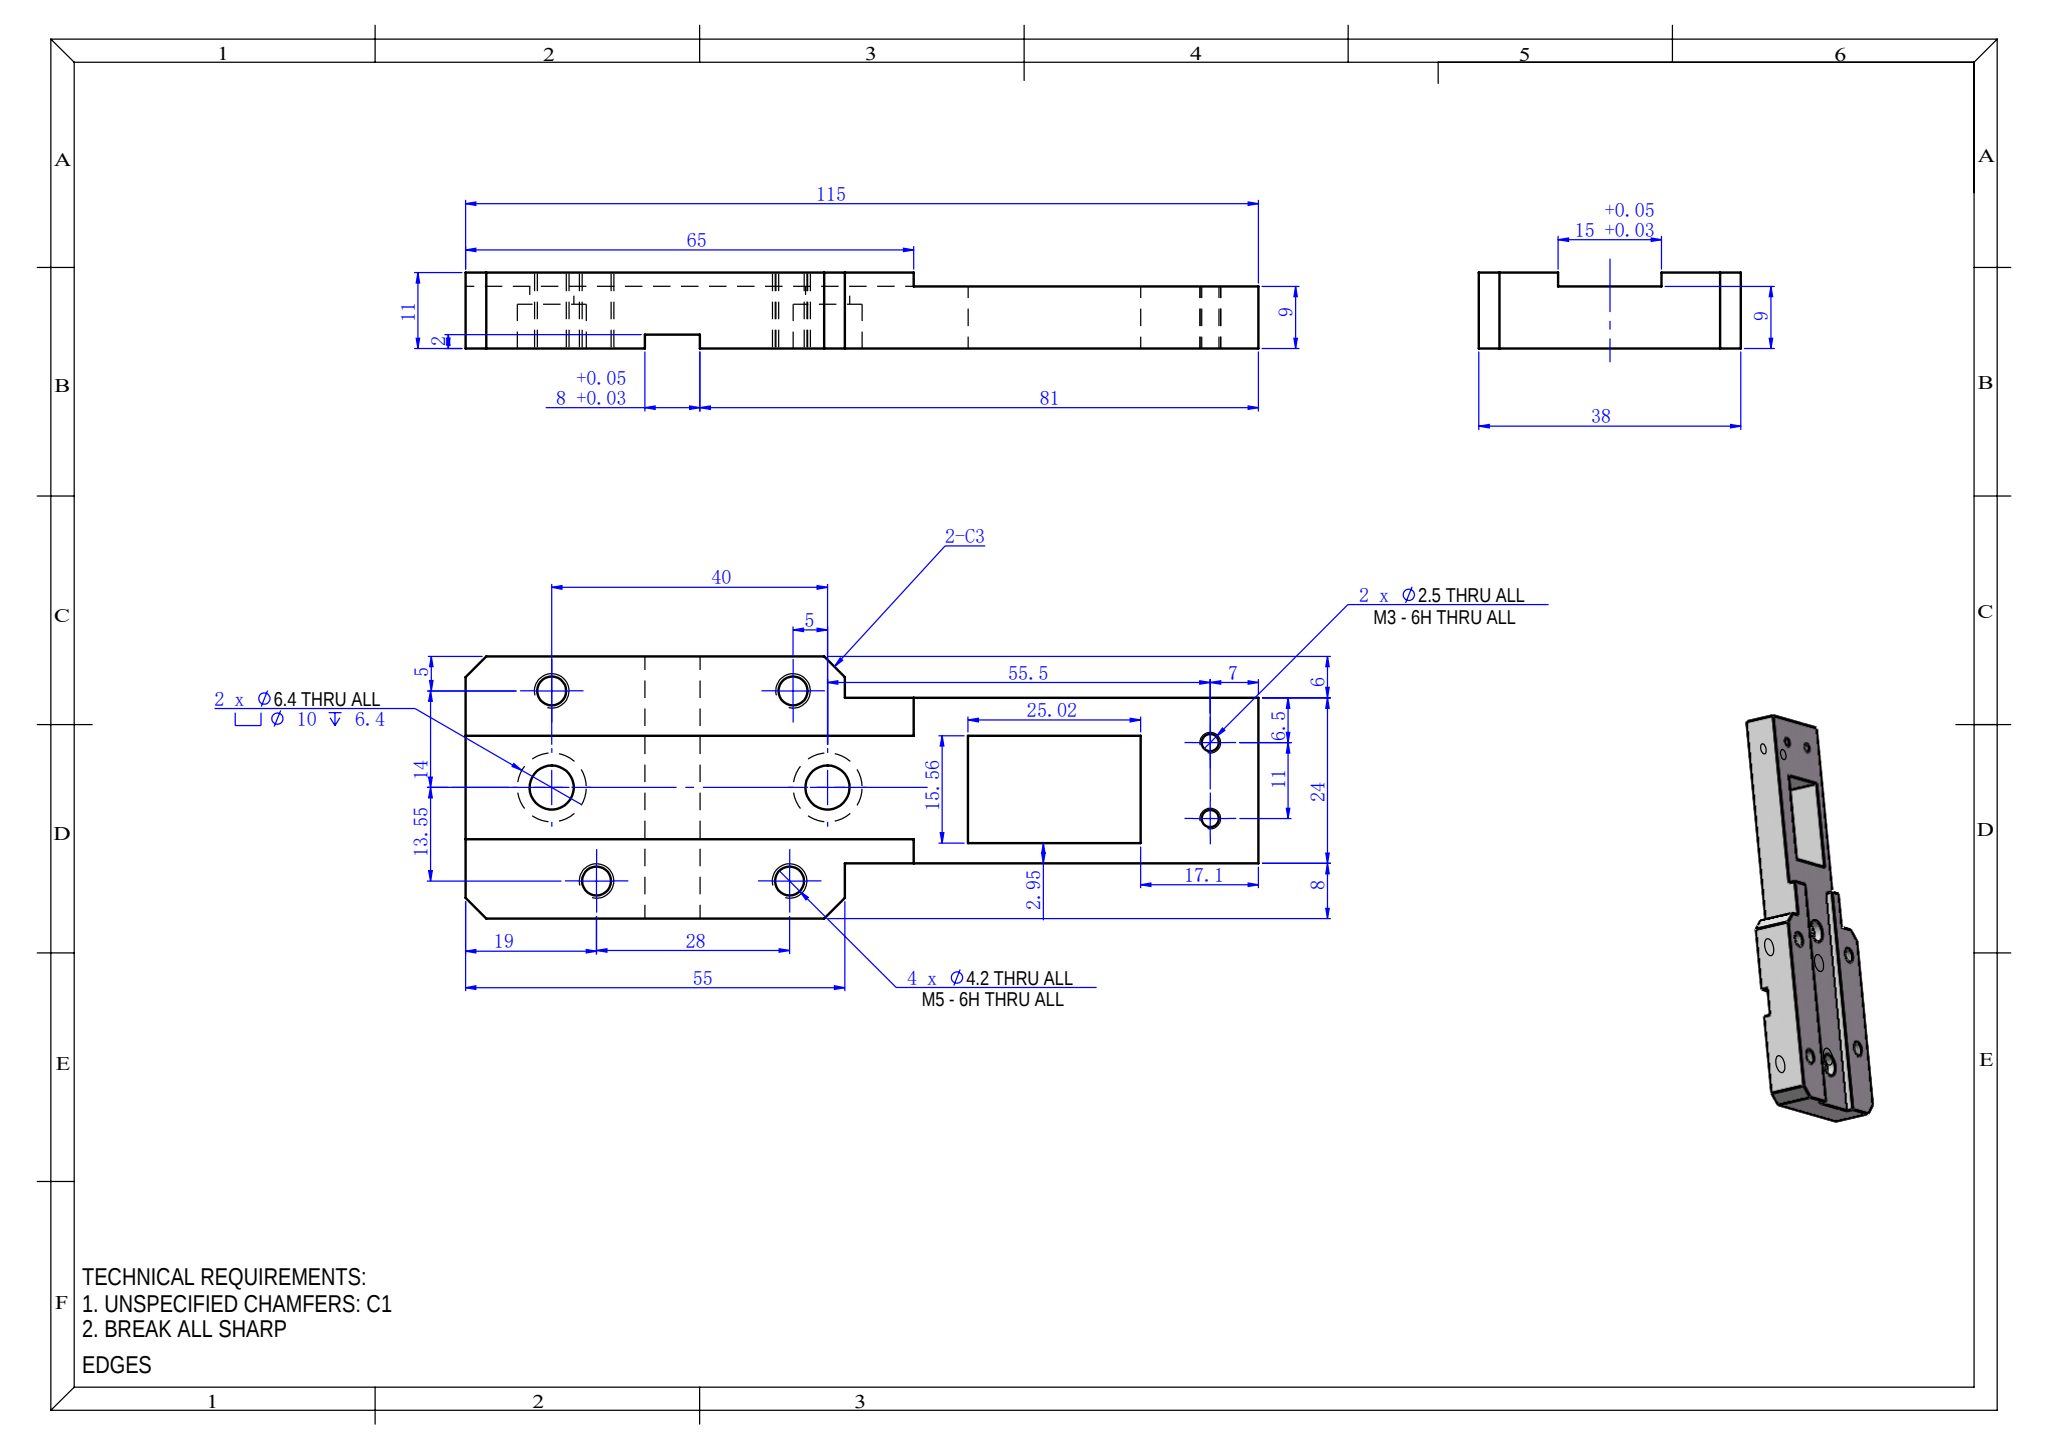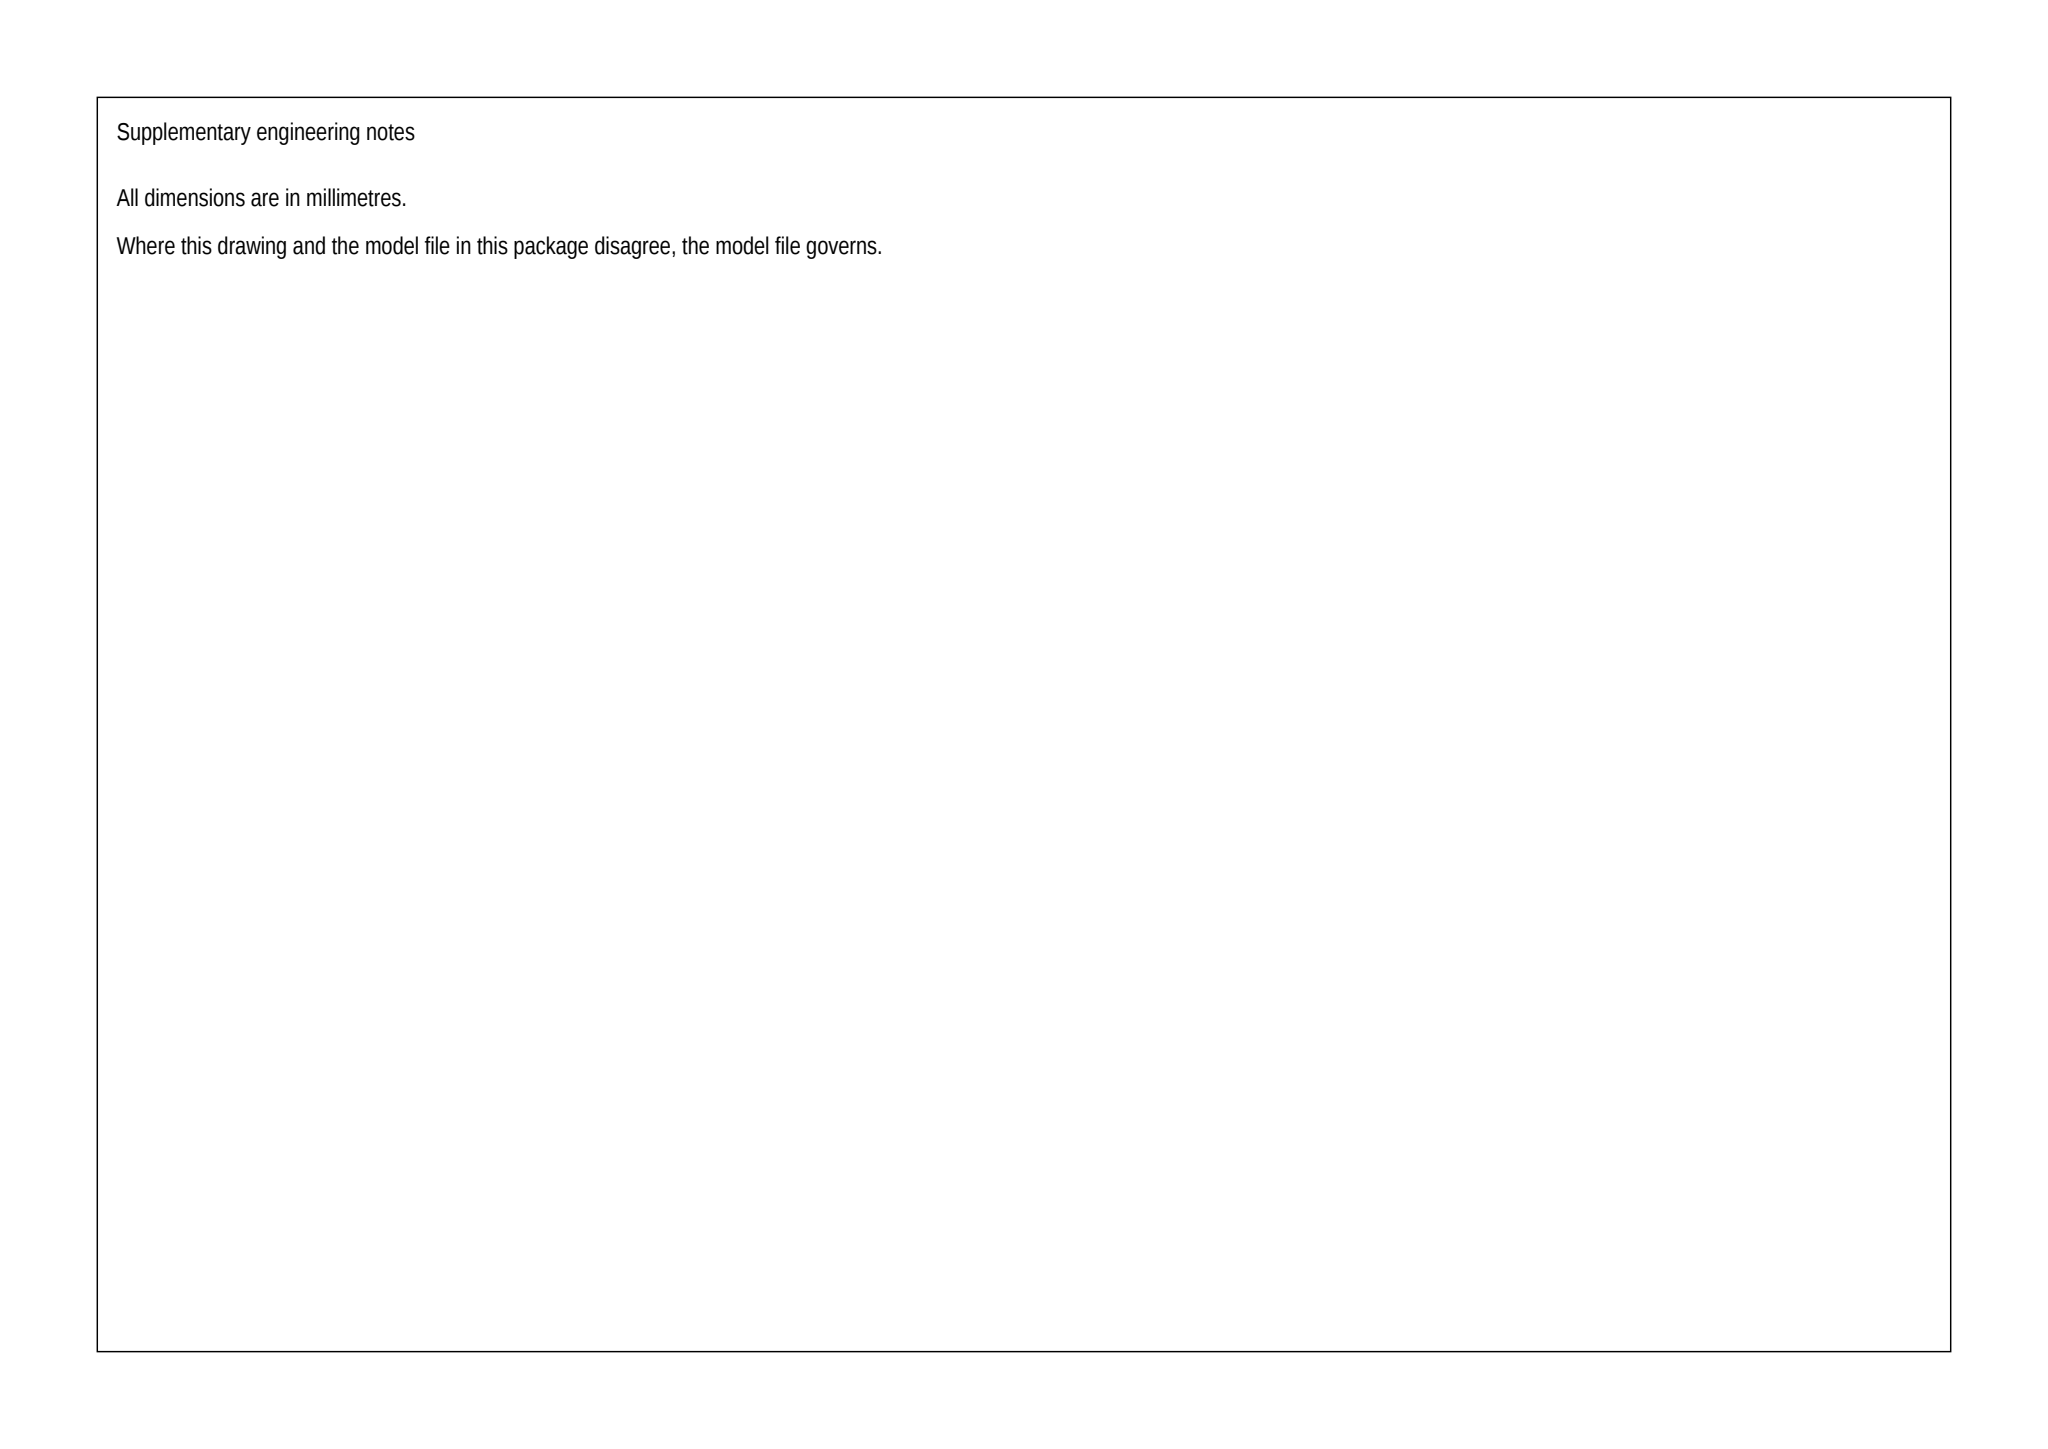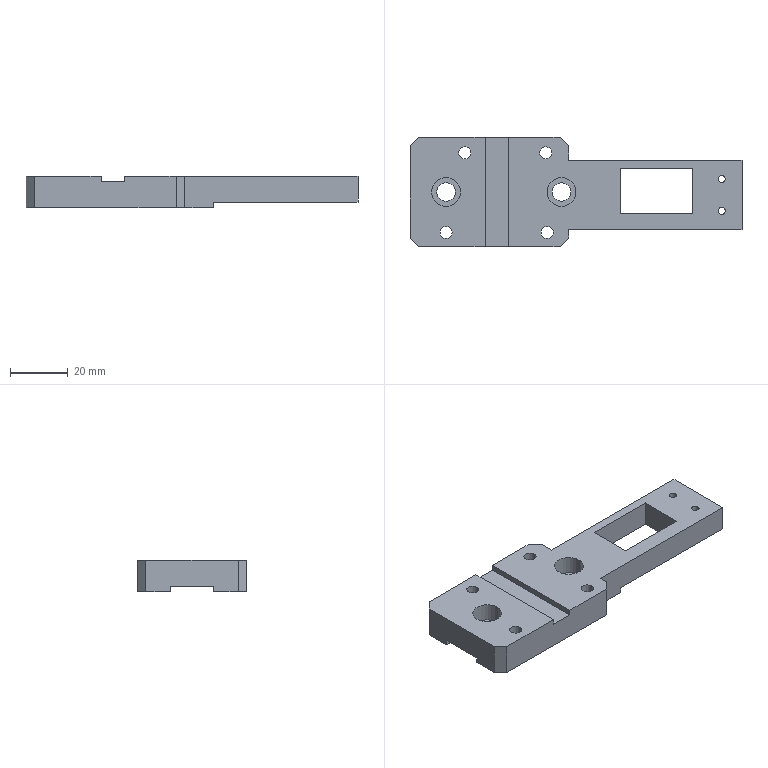Part | SolidWorks | mm | 1 solid | 50 faces | box 115 x 38 x 11 mm | volume 28299 mm3 | plane 30 | cylinder 20 | commonest cylinder face diameters 4.2 x8 10 x4 6.4 x4 2.5 x4
Drawing notes:
SLOT 15 +0.05/+0.03 WIDE x 2 DP IN TOP FACE, FULL 115 LG | from the solid: y-planes 11.5 & 26.5 (15 wide, CL y=19); floor z=9.0 vs top z=11.0; runs full bbox x=115
BOTTOM BOSS 8 WIDE x 2 HIGH, 26 FROM LEFT END FACE | from the solid: x-planes 26.0 & 34.0 (8 wide) from x=0 end face; z=0.0 faces up to main bottom z=2.0, OAH 11
POCKET 25.02 x 15.56 THRU, 7 DP FROM SLOT FLOOR | from the solid: x-planes 72.88/97.9 = 25.02; y-planes 11.49/27.05 = 15.56; no z-plane between slot floor z=9 and z=2
2 x Ø6.4 THRU ALL, CBORE Ø10 DP 6.4 FROM TOP FACE | from the solid: Coaxial cyls at (12.5,19) & (52.5,19): Ø10 L6.4 z=11 to 4.6, Ø6.4 L2.6 z=4.6 to 2; z-planes 4.6 = CBORE floors
build123d program:
from build123d import *

# Parameters (mm, degrees)
SKETCH1_W                                       = 115
SKETCH1_H                                       = 38
BOSS_EXTRUDE1_DEPTH                             = 11
SKETCH3_W                                       = 2
SKETCH3_H                                       = 15
CUT_EXTRUDE2_DEPTH                              = 125.887
M5_TAPPED_HOLE1_D                               = 4.2
SKETCH6_W                                       = 50
SKETCH6_H                                       = 2
CUT_EXTRUDE3_DEPTH                              = 96.654
M3_TAPPED_HOLE1_D                               = 2.5
SKETCH9_W                                       = 60
SKETCH9_H                                       = 8
SKETCH9_H_2                                     = 6
CUT_EXTRUDE4_DEPTH                              = 100.783
CHAMFER1_SIZE                                   = 3
M6_HEX_SOCKET_HEAD_CAP_SCREW_CBORE1_D           = 6.4
M6_HEX_SOCKET_HEAD_CAP_SCREW_CBORE1_CBORE_D     = 10
M6_HEX_SOCKET_HEAD_CAP_SCREW_CBORE1_CBORE_DEPTH = 6.4
SKETCH14_W                                      = 8
SKETCH14_H                                      = 2
CUT_EXTRUDE5_DEPTH                              = 96.654
SKETCH15_W                                      = 25.024
SKETCH15_H                                      = 15.56
CUT_EXTRUDE6_DEPTH                              = 22


with BuildPart() as part:
    # Sketch1 → Boss-Extrude1 (new body)
    with BuildSketch(Plane.XY):
        with Locations((29.59, 28.443)):
            Rectangle(SKETCH1_W, SKETCH1_H)
    extrude(amount=BOSS_EXTRUDE1_DEPTH)

    # Sketch3 → Cut-Extrude2 (cut, through all)
    with BuildSketch(Plane(origin=(87.09, 0, 0), x_dir=(0, 0, -1), z_dir=(1, 0, 0))):
        with Locations((-1, 28.443)):
            Rectangle(SKETCH3_W, SKETCH3_H)
    extrude(amount=-CUT_EXTRUDE2_DEPTH, mode=Mode.SUBTRACT)

    # M5 Tapped Hole1 (through all)
    with Locations(Plane.XY.offset(11)):
        with Locations((-8.91, 41.993), (19.09, 41.993), (19.59, 14.443), (-15.41, 14.443)):
            Hole(M5_TAPPED_HOLE1_D / 2)

    # Sketch6 → Cut-Extrude3 (cut, through all)
    with BuildSketch(Plane(origin=(0, 9.443, 0), x_dir=(-1, 0, 0), z_dir=(0, -1, 0))):
        with Locations((-62.09, -1)):
            Rectangle(SKETCH6_W, SKETCH6_H)
    extrude(amount=-CUT_EXTRUDE3_DEPTH, mode=Mode.SUBTRACT)

    # M3 Tapped Hole1 (through all)
    with Locations(Plane.XY.offset(11)):
        with Locations((80.09, 21.943), (80.09, 32.943)):
            Hole(M3_TAPPED_HOLE1_D / 2)

    # Sketch9 → Cut-Extrude4 (cut, through all)
    with BuildSketch(Plane.XY.offset(11)):
        with Locations((57.09, 43.443)):
            Rectangle(SKETCH9_W, SKETCH9_H)
        with Locations((57.09, 12.443)):
            Rectangle(SKETCH9_W, SKETCH9_H_2)
    extrude(amount=-CUT_EXTRUDE4_DEPTH, mode=Mode.SUBTRACT)

    # Chamfer1
    chamfer1_edges = [part.edges().sort_by_distance(p)[0] for p in [
        (27.09, 9.443, 5.5),
        (-27.91, 9.443, 5.5),
        (-27.91, 47.443, 5.5),
        (27.09, 47.443, 5.5),
    ]]
    chamfer(chamfer1_edges, length=CHAMFER1_SIZE)

    # M6 Hex Socket Head Cap Screw CBORE1 (through all)
    with Locations(Plane.XY.offset(11)):
        with Locations((24.59, 28.443), (-15.41, 28.443)):
            CounterBoreHole(M6_HEX_SOCKET_HEAD_CAP_SCREW_CBORE1_D / 2, M6_HEX_SOCKET_HEAD_CAP_SCREW_CBORE1_CBORE_D / 2, M6_HEX_SOCKET_HEAD_CAP_SCREW_CBORE1_CBORE_DEPTH)

    # Sketch14 → Cut-Extrude5 (cut, through all)
    with BuildSketch(Plane(origin=(0, 47.443, 0), x_dir=(1, 0, 0), z_dir=(0, 1, 0))):
        with Locations((2.09, -10)):
            Rectangle(SKETCH14_W, SKETCH14_H)
    extrude(amount=-CUT_EXTRUDE5_DEPTH, mode=Mode.SUBTRACT)

    # Sketch15 → Cut-Extrude6 (cut)
    with BuildSketch(Plane(origin=(0, 0, 2), x_dir=(-1, 0, 0), z_dir=(0, 0, -1))):
        with Locations((-57.481, 28.716)):
            Rectangle(SKETCH15_W, SKETCH15_H)
    extrude(amount=-CUT_EXTRUDE6_DEPTH, mode=Mode.SUBTRACT)


solid = part.part